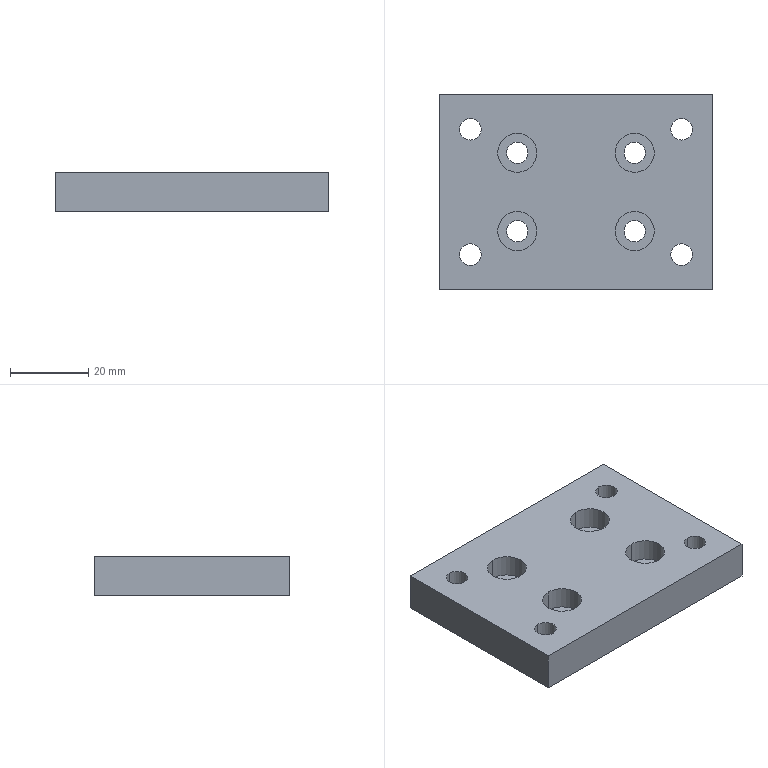Component | SolidWorks | 01-15MarkingMachineMountingSeatPlate2-1 | 1 solid | 46 faces | box 70 x 50 x 10 mm | volume 30776 mm3 | cylinder 32 | plane 14 | commonest cylinder face diameters 5.5 x16 9.5 x8 10 x8 | material A3 Steel
build123d program:
from build123d import *

# Parameters (mm, degrees)
SKETCH1_W                                          = 50
SKETCH1_H                                          = 70
BOSS_EXTRUDE1_DEPTH                                = 10
HOLE_SIZE_ACCORDING_TO_TYPE_1_OF_HEXAG_D           = 5.5
HOLE_SIZE_ACCORDING_TO_TYPE_1_OF_HEXAG_CBORE_D     = 10
HOLE_SIZE_ACCORDING_TO_TYPE_1_OF_HEXAG_CBORE_DEPTH = 5.7
HOLE_SIZE_ACCORDING_TO_TYPE_3_OF_HEXAG_D           = 5.5
HOLE_SIZE_ACCORDING_TO_TYPE_3_OF_HEXAG_CBORE_D     = 9.5
HOLE_SIZE_ACCORDING_TO_TYPE_3_OF_HEXAG_CBORE_DEPTH = 5.7


with BuildPart() as part:
    # Sketch1 → Boss-Extrude1 (new body)
    with BuildSketch(Plane.XY):
        Rectangle(SKETCH1_W, SKETCH1_H)
    extrude(amount=BOSS_EXTRUDE1_DEPTH)

    # Hole Size _According to_ Type 1 of Hexag (through all)
    with Locations(Plane(origin=(-10, 15, 10), x_dir=(1, 0, 0), z_dir=(0, 0, 1))):
        with Locations((0, 0), (20, 0), (20, -30), (0, -30)):
            CounterBoreHole(HOLE_SIZE_ACCORDING_TO_TYPE_1_OF_HEXAG_D / 2, HOLE_SIZE_ACCORDING_TO_TYPE_1_OF_HEXAG_CBORE_D / 2, HOLE_SIZE_ACCORDING_TO_TYPE_1_OF_HEXAG_CBORE_DEPTH)

    # Hole Size _According to_ Type 3 of Hexag (through all)
    with Locations(Plane(origin=(16, 27, 0), x_dir=(-1, 0, 0), z_dir=(0, 0, -1))):
        with Locations((0, 0), (32, 0), (32, -54), (0, -54)):
            CounterBoreHole(HOLE_SIZE_ACCORDING_TO_TYPE_3_OF_HEXAG_D / 2, HOLE_SIZE_ACCORDING_TO_TYPE_3_OF_HEXAG_CBORE_D / 2, HOLE_SIZE_ACCORDING_TO_TYPE_3_OF_HEXAG_CBORE_DEPTH)


solid = part.part

# Placed as in the assembly
solid = solid.moved(Location((-179.532, 2.41, -140), (0, 0, 90)))